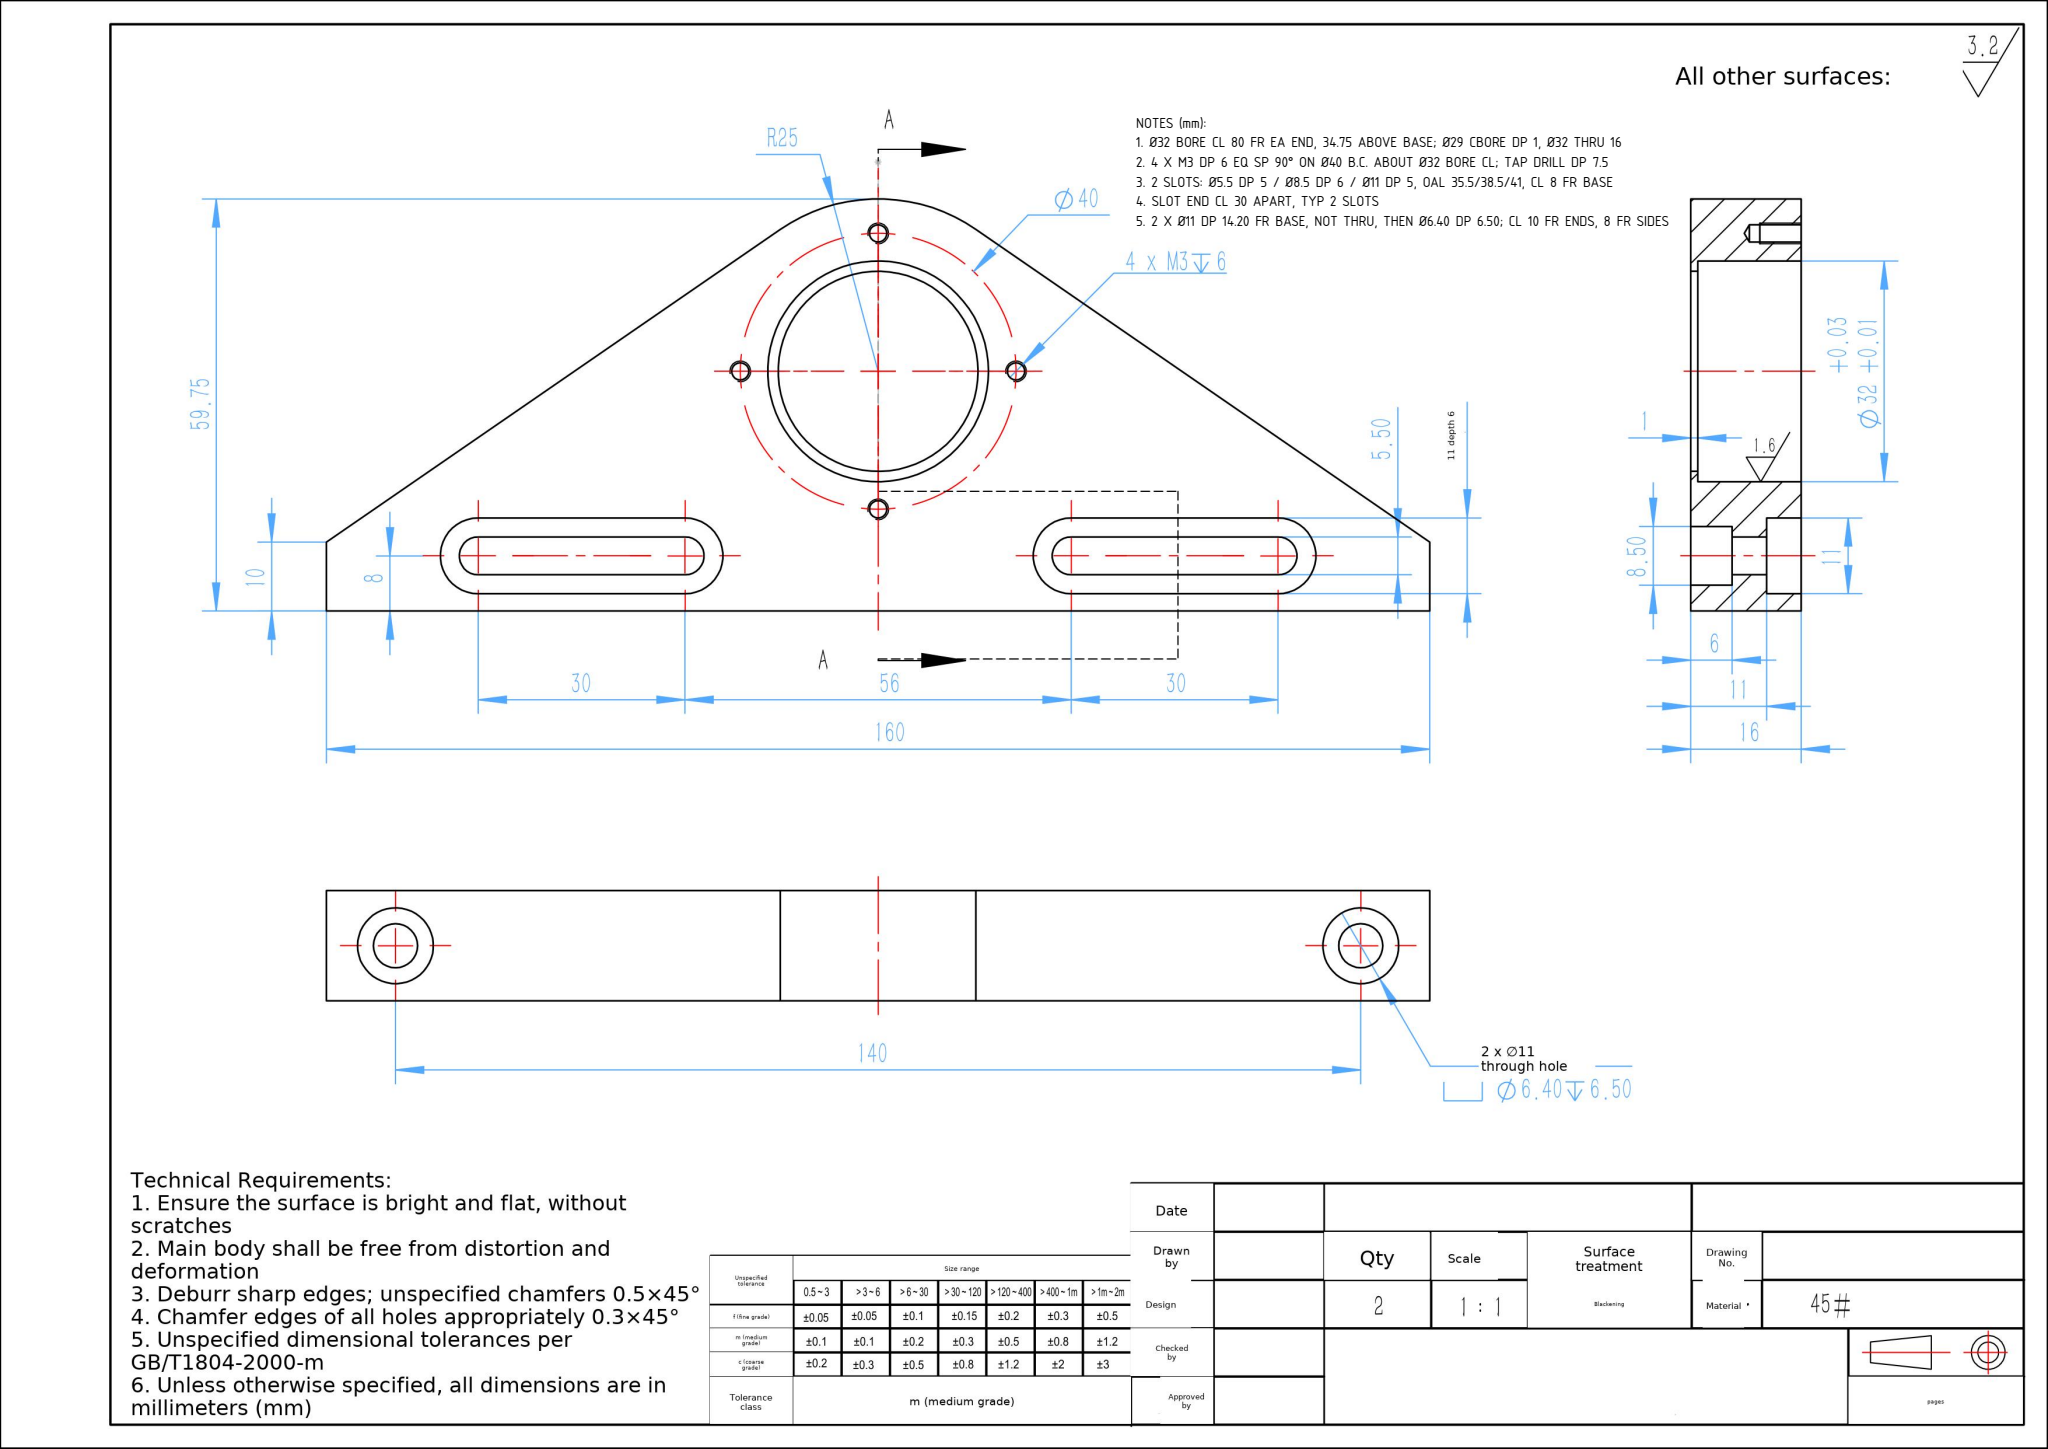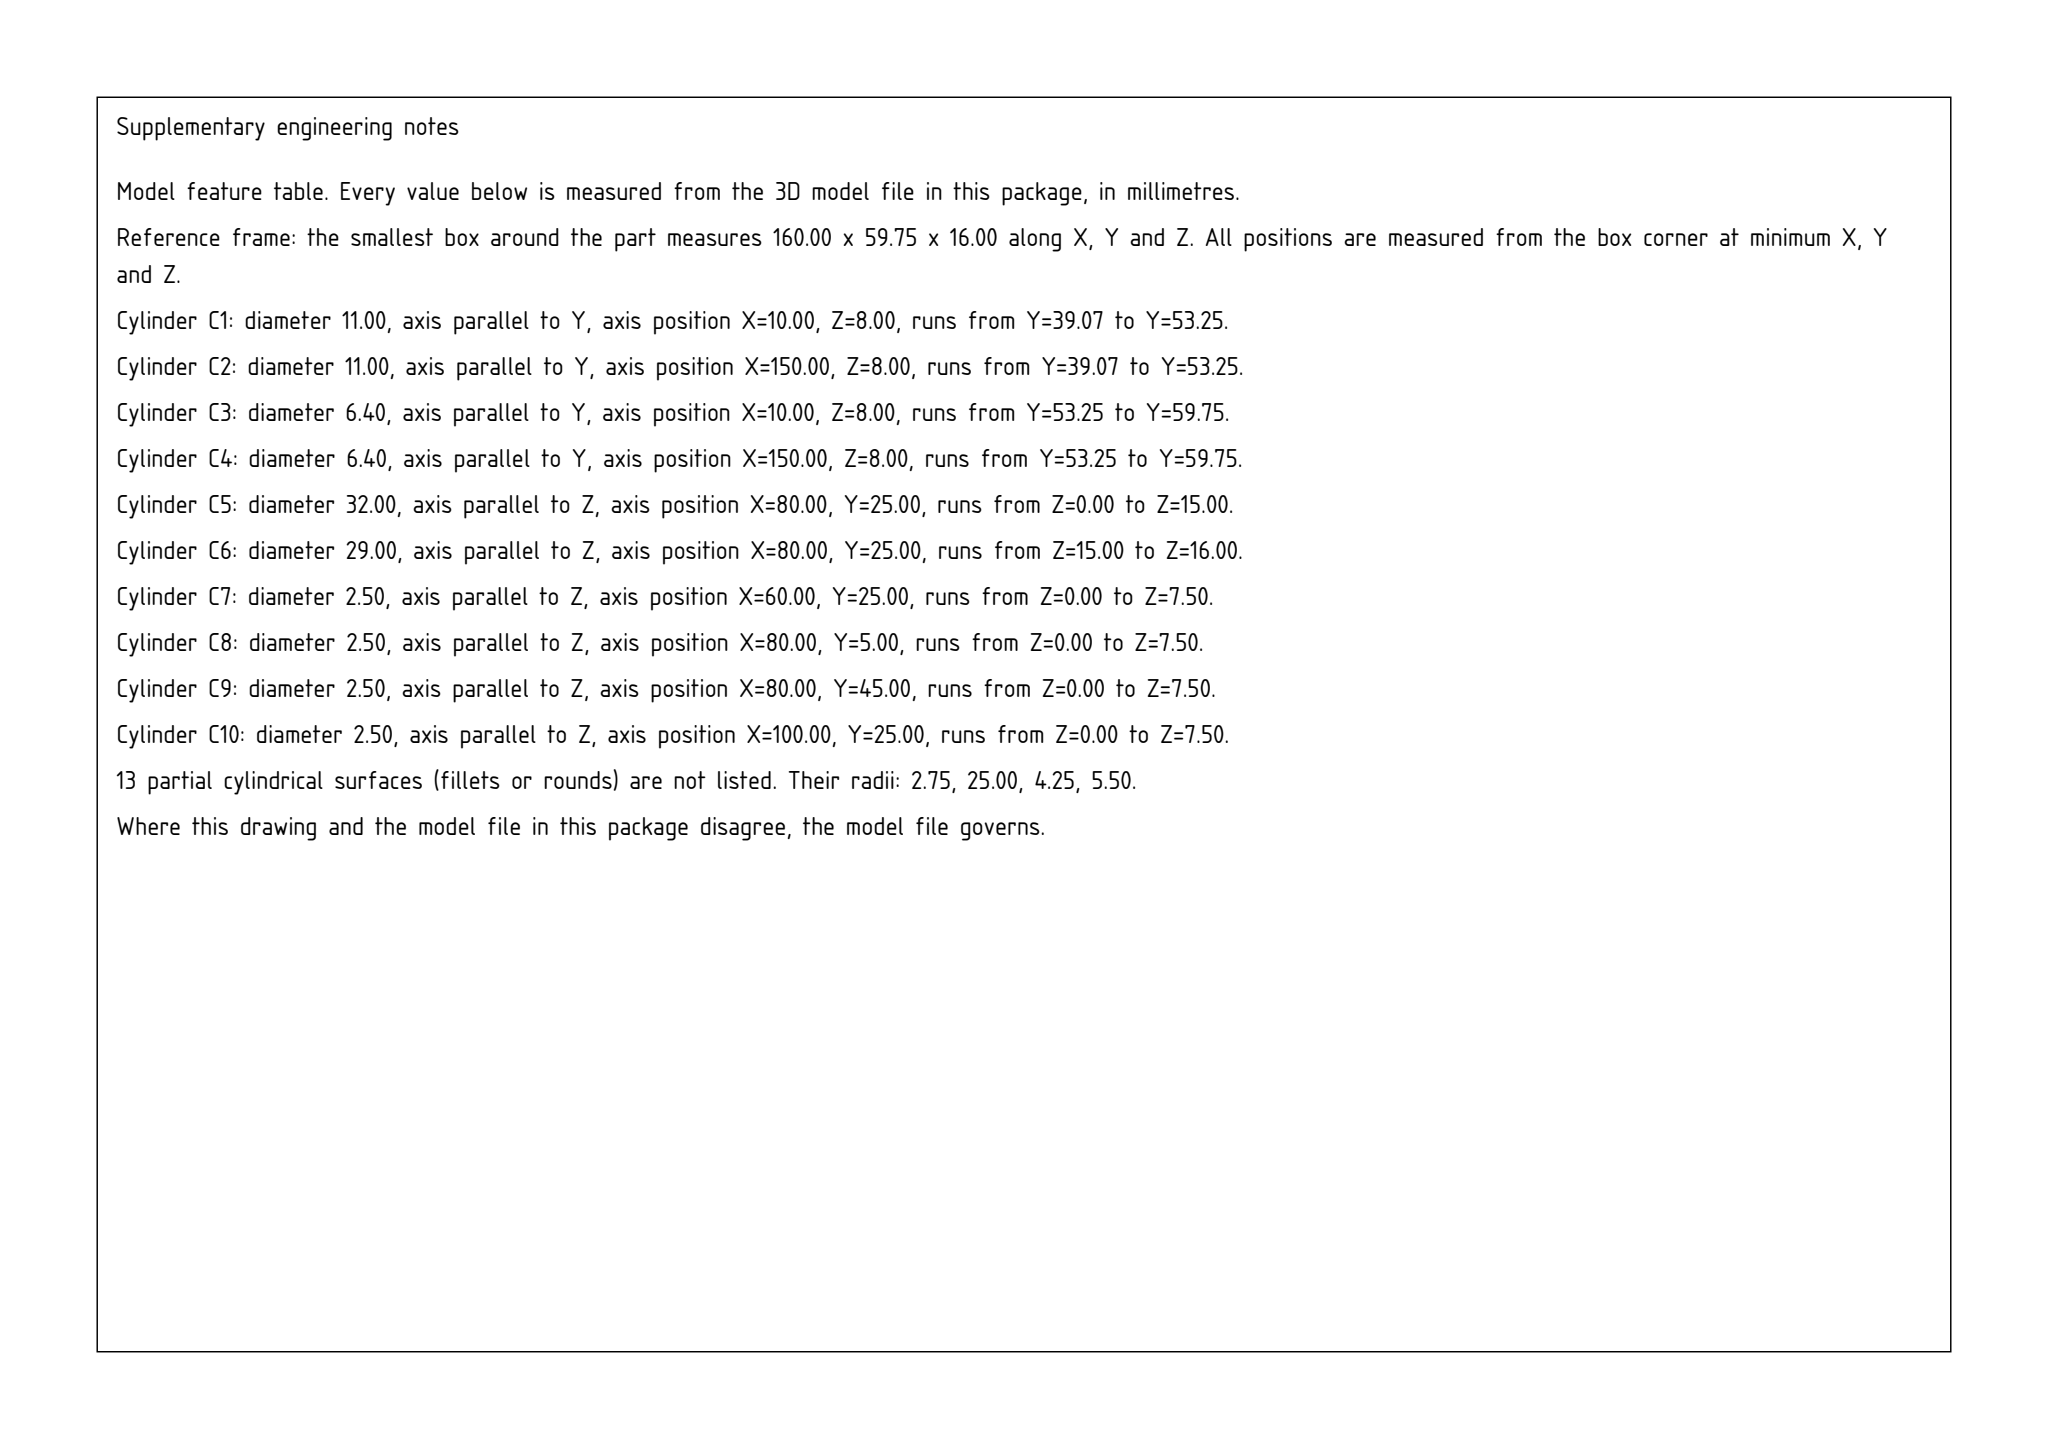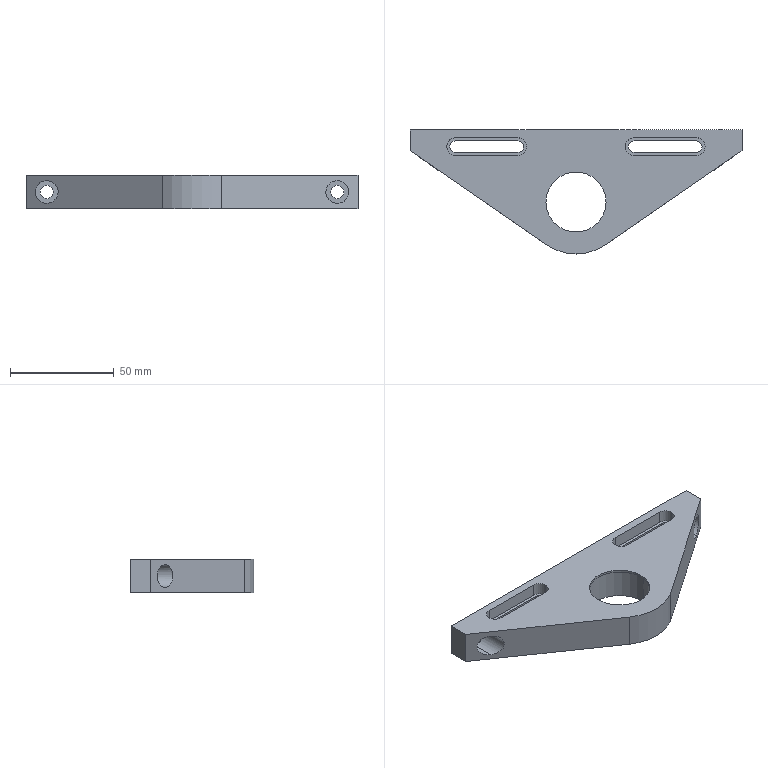Part | SolidWorks | mm | 1 solid | 73 faces | box 160 x 59.75 x 16 mm | volume 70133 mm3 | cylinder 39 | plane 26 | cone 8 | commonest cylinder face diameters 11 x10 2.5 x8 8.5 x6 5.5 x6 6.4 x4 32 x2 29 x2 50 x1
Drawing notes:
Ø32 BORE CL 80 FR EA END, 34.75 ABOVE BASE; Ø29 CBORE DP 1, Ø32 THRU 16 | from the solid: z-cyls at (80,25): Ø29 L=1, Ø32 L=15, Ø50 L=16; bbox 160x59.75x16, 59.75-25=34.75
4 X M3 DP 6 EQ SP 90° ON Ø40 B.C. ABOUT Ø32 BORE CL; TAP DRILL DP 7.5 | from the solid: Ø2.5 z-holes at (60,25),(80,5),(80,45),(100,25) = R20 about (80,25), L=7.5
2 SLOTS: Ø5.5 DP 5 / Ø8.5 DP 6 / Ø11 DP 5, OAL 35.5/38.5/41, CL 8 FR BASE | from the solid: slot end cyls y=51.75 (59.75-51.75=8); dias 11 L5, 8.5 L6, 5.5 L5; z planes 0/5/10/15
SLOT END CL 30 APART, TYP 2 SLOTS | from the solid: end cyl axes x=22/52 and x=108/138, 30 apart
2 X Ø11 DP 14.20 FR BASE, NOT THRU, THEN Ø6.40 DP 6.50; CL 10 FR ENDS, 8 FR SIDES | from the solid: y-axis Ø11 L=14.2 (10.39 cut by chamfer) and coaxial Ø6.4 L=6.5 at x=10 & 150, z=8; 20.70<59.75
build123d program:
from build123d import *

# Parameters (mm, degrees)
SKETCH1_R                                = 14.5
BOSS_EXTRUDE1_DEPTH                      = 8
SKETCH2_R                                = 16
CUT_EXTRUDE1_DEPTH                       = 15
HOLE_SIZE_ACCORDING_TO_TYPE_1_OF_2_COUNT = 2
HOLE_SIZE_ACCORDING_TO_TYPE_1_OF_2_PITCH = 140
M3_TAPPED_HOLE1_D                        = 2.5
M3_TAPPED_HOLE1_DEPTH                    = 7.5
M3_TAPPED_HOLE1_TIP                      = 0.7511
CUT_EXTRUDE3_DEPTH                       = 102.124
CUT_EXTRUDE4_DEPTH                       = 6
CUT_EXTRUDE5_DEPTH                       = 5


with BuildPart() as part:
    # Sketch1 → Boss-Extrude1 (new, symmetric)
    with BuildSketch(Plane.XY):
        with BuildLine():
            Line((80, 0), (-80, 0))
            Line((-80, 0), (-80, -10))
            Line((-80, -10), (-14.182, -55.338))
            ThreePointArc((-14.182, -55.338), (0, -59.75), (14.182, -55.338))
            Line((14.182, -55.338), (80, -10))
            Line((80, -10), (80, 0))
        make_face()
        with Locations((0, -34.75)):
            Circle(SKETCH1_R, mode=Mode.SUBTRACT)
    extrude(amount=BOSS_EXTRUDE1_DEPTH, both=True)

    # Sketch2 → Cut-Extrude1 (cut)
    with BuildSketch(Plane.XY.offset(-8)):
        with Locations((0, -34.75)):
            Circle(SKETCH2_R)
    extrude(amount=CUT_EXTRUDE1_DEPTH, mode=Mode.SUBTRACT)

    # Sketch3 → Hole Size _ according to_ type 1 of Hexa (revolve, cut)
    with BuildSketch(Plane(origin=(-70, 0, 0), x_dir=(0, 0, 1), z_dir=(1, 0, 0))):
        Polygon((0, 0), (0, 59.75), (5.5, 59.75), (5.5, 6.5), (3.2, 6.5), (3.2, 0), align=None)
    hole_size_according_to_type_1_of_hexa = revolve(axis=Axis((-70, 6.35, 0), (0, -1, 0)), mode=Mode.SUBTRACT)

    # Hole Size _ according to_ type 1 of  2: Hole Size _ according to_ type 1 of Hexa ×2
    with Locations(*[(i * HOLE_SIZE_ACCORDING_TO_TYPE_1_OF_2_PITCH, 0, 0) for i in range(1, HOLE_SIZE_ACCORDING_TO_TYPE_1_OF_2_COUNT)]):
        add(hole_size_according_to_type_1_of_hexa, mode=Mode.SUBTRACT)

    # M3 Tapped Hole1
    with Locations(Plane(origin=(0, 0, -8), x_dir=(1, 0, 0), z_dir=(0, 0, -1))):
        with Locations((0, 14.75), (-20, 34.75), (0, 54.75), (20, 34.75)):
            Hole(M3_TAPPED_HOLE1_D / 2, depth=M3_TAPPED_HOLE1_DEPTH)
            with Locations((0, 0, -(M3_TAPPED_HOLE1_DEPTH + M3_TAPPED_HOLE1_TIP / 2))):  # 118° drill point
                Cone(0, M3_TAPPED_HOLE1_D / 2, M3_TAPPED_HOLE1_TIP, mode=Mode.SUBTRACT)

    # Sketch8 → Cut-Extrude3 (cut, through all)
    with BuildSketch(Plane.XY.offset(8)):
        with BuildLine():
            Line((-58, -5.25), (-28, -5.25))
            ThreePointArc((-28, -5.25), (-25.25, -8), (-28, -10.75))
            Line((-28, -10.75), (-58, -10.75))
            ThreePointArc((-58, -10.75), (-60.75, -8), (-58, -5.25))
        make_face()
    cut_extrude3 = extrude(amount=-CUT_EXTRUDE3_DEPTH, mode=Mode.SUBTRACT)

    # Sketch9 → Cut-Extrude4 (cut)
    with BuildSketch(Plane.XY.offset(8)):
        with BuildLine():
            Line((-58, -3.75), (-28, -3.75))
            ThreePointArc((-28, -3.75), (-23.75, -8), (-28, -12.25))
            Line((-28, -12.25), (-58, -12.25))
            ThreePointArc((-58, -12.25), (-62.25, -8), (-58, -3.75))
        make_face()
    cut_extrude4 = extrude(amount=-CUT_EXTRUDE4_DEPTH, mode=Mode.SUBTRACT)

    # Sketch10 → Cut-Extrude5 (cut)
    with BuildSketch(Plane(origin=(0, 0, -8), x_dir=(-1, 0, 0), z_dir=(0, 0, -1))):
        with BuildLine():
            Line((28, -2.5), (58, -2.5))
            ThreePointArc((58, -2.5), (63.5, -8), (58, -13.5))
            Line((58, -13.5), (28, -13.5))
            ThreePointArc((28, -13.5), (22.5, -8), (28, -2.5))
        make_face()
    cut_extrude5 = extrude(amount=-CUT_EXTRUDE5_DEPTH, mode=Mode.SUBTRACT)

    # Mirror1: Cut-Extrude3, Cut-Extrude4, Cut-Extrude5 across plane
    add(cut_extrude3.mirror(Plane(origin=(0, 0, 0), x_dir=(0, 0, 1), z_dir=(1, 0, 0))), mode=Mode.SUBTRACT)
    add(cut_extrude4.mirror(Plane(origin=(0, 0, 0), x_dir=(0, 0, 1), z_dir=(1, 0, 0))), mode=Mode.SUBTRACT)
    add(cut_extrude5.mirror(Plane(origin=(0, 0, 0), x_dir=(0, 0, 1), z_dir=(1, 0, 0))), mode=Mode.SUBTRACT)


solid = part.part